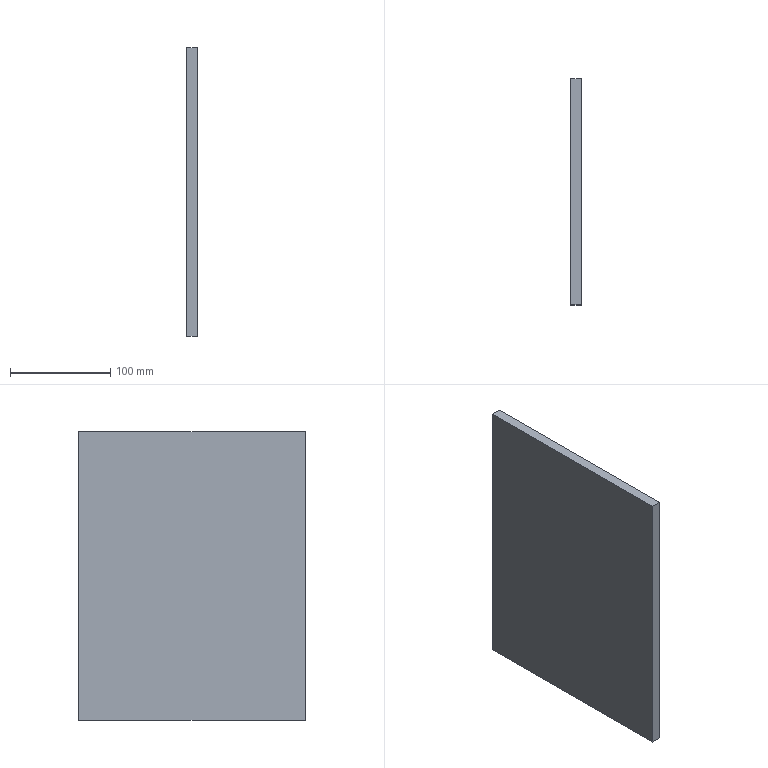Component | SolidWorks | Cover2-1 | 1 solid | 6 faces | box 10 x 226 x 288 mm | volume 650880 mm3 | plane 6 | material Plain Carbon Steel
STEP:
#1=COLOUR_RGB('',0.7922,0.8196,0.9333);
#2=FILL_AREA_STYLE_COLOUR('',#1);
#3=FILL_AREA_STYLE('',(#2));
#4=SURFACE_STYLE_FILL_AREA(#3);
#5=SURFACE_SIDE_STYLE('',(#4));
#6=SURFACE_STYLE_USAGE(.BOTH.,#5);
#7=PRESENTATION_STYLE_ASSIGNMENT((#6));
#8=CARTESIAN_POINT('',(88.212,53.911,76.893));
#9=VERTEX_POINT('',#8);
#10=CARTESIAN_POINT('',(88.212,53.911,65.555));
#11=VERTEX_POINT('',#10);
#12=CARTESIAN_POINT('',(88.212,53.911,65.555));
#13=DIRECTION('',(0.,-0.,-1.));
#14=VECTOR('',#13,39.37);
#15=LINE('',#12,#14);
#16=EDGE_CURVE('',#9,#11,#15,.T.);
#17=ORIENTED_EDGE('',*,*,#16,.F.);
#18=CARTESIAN_POINT('',(88.605,53.911,76.893));
#19=VERTEX_POINT('',#18);
#20=CARTESIAN_POINT('',(88.605,53.911,76.893));
#21=DIRECTION('',(-1.,-0.,0.));
#22=VECTOR('',#21,39.37);
#23=LINE('',#20,#22);
#24=EDGE_CURVE('',#19,#9,#23,.T.);
#25=ORIENTED_EDGE('',*,*,#24,.F.);
#26=CARTESIAN_POINT('',(88.605,53.911,65.555));
#27=VERTEX_POINT('',#26);
#28=CARTESIAN_POINT('',(88.605,53.911,65.555));
#29=DIRECTION('',(0.,-0.,-1.));
#30=VECTOR('',#29,39.37);
#31=LINE('',#28,#30);
#32=EDGE_CURVE('',#19,#27,#31,.T.);
#33=ORIENTED_EDGE('',*,*,#32,.T.);
#34=CARTESIAN_POINT('',(88.605,53.911,65.555));
#35=DIRECTION('',(-1.,-0.,0.));
#36=VECTOR('',#35,39.37);
#37=LINE('',#34,#36);
#38=EDGE_CURVE('',#27,#11,#37,.T.);
#39=ORIENTED_EDGE('',*,*,#38,.T.);
#40=EDGE_LOOP('',(#17,#25,#33,#39));
#41=FACE_OUTER_BOUND('',#40,.T.);
#42=CARTESIAN_POINT('',(88.605,53.911,65.555));
#43=DIRECTION('',(-0.,1.,-0.));
#44=DIRECTION('',(0.,-0.,-1.));
#45=AXIS2_PLACEMENT_3D('',#42,#43,#44);
#46=PLANE('',#45);
#47=ADVANCED_FACE('',(#41),#46,.T.);
#48=CARTESIAN_POINT('',(88.212,45.014,76.893));
#49=VERTEX_POINT('',#48);
#50=CARTESIAN_POINT('',(88.212,45.014,76.893));
#51=DIRECTION('',(-0.,1.,0.));
#52=VECTOR('',#51,39.37);
#53=LINE('',#50,#52);
#54=EDGE_CURVE('',#49,#9,#53,.T.);
#55=ORIENTED_EDGE('',*,*,#54,.F.);
#56=CARTESIAN_POINT('',(88.605,45.014,76.893));
#57=VERTEX_POINT('',#56);
#58=CARTESIAN_POINT('',(88.605,45.014,76.893));
#59=DIRECTION('',(-1.,-0.,0.));
#60=VECTOR('',#59,39.37);
#61=LINE('',#58,#60);
#62=EDGE_CURVE('',#57,#49,#61,.T.);
#63=ORIENTED_EDGE('',*,*,#62,.F.);
#64=CARTESIAN_POINT('',(88.605,45.014,76.893));
#65=DIRECTION('',(-0.,1.,0.));
#66=VECTOR('',#65,39.37);
#67=LINE('',#64,#66);
#68=EDGE_CURVE('',#57,#19,#67,.T.);
#69=ORIENTED_EDGE('',*,*,#68,.T.);
#70=ORIENTED_EDGE('',*,*,#24,.T.);
#71=EDGE_LOOP('',(#55,#63,#69,#70));
#72=FACE_OUTER_BOUND('',#71,.T.);
#73=CARTESIAN_POINT('',(88.605,45.014,76.893));
#74=DIRECTION('',(0.,0.,1.));
#75=DIRECTION('',(-0.,1.,0.));
#76=AXIS2_PLACEMENT_3D('',#73,#74,#75);
#77=PLANE('',#76);
#78=ADVANCED_FACE('',(#72),#77,.T.);
#79=CARTESIAN_POINT('',(88.212,45.014,65.555));
#80=VERTEX_POINT('',#79);
#81=CARTESIAN_POINT('',(88.212,45.014,65.555));
#82=DIRECTION('',(-0.,0.,1.));
#83=VECTOR('',#82,39.37);
#84=LINE('',#81,#83);
#85=EDGE_CURVE('',#80,#49,#84,.T.);
#86=ORIENTED_EDGE('',*,*,#85,.F.);
#87=CARTESIAN_POINT('',(88.605,45.014,65.555));
#88=VERTEX_POINT('',#87);
#89=CARTESIAN_POINT('',(88.605,45.014,65.555));
#90=DIRECTION('',(-1.,-0.,0.));
#91=VECTOR('',#90,39.37);
#92=LINE('',#89,#91);
#93=EDGE_CURVE('',#88,#80,#92,.T.);
#94=ORIENTED_EDGE('',*,*,#93,.F.);
#95=CARTESIAN_POINT('',(88.605,45.014,65.555));
#96=DIRECTION('',(-0.,0.,1.));
#97=VECTOR('',#96,39.37);
#98=LINE('',#95,#97);
#99=EDGE_CURVE('',#88,#57,#98,.T.);
#100=ORIENTED_EDGE('',*,*,#99,.T.);
#101=ORIENTED_EDGE('',*,*,#62,.T.);
#102=EDGE_LOOP('',(#86,#94,#100,#101));
#103=FACE_OUTER_BOUND('',#102,.T.);
#104=CARTESIAN_POINT('',(88.605,45.014,65.555));
#105=DIRECTION('',(0.,-1.,0.));
#106=DIRECTION('',(-0.,0.,1.));
#107=AXIS2_PLACEMENT_3D('',#104,#105,#106);
#108=PLANE('',#107);
#109=ADVANCED_FACE('',(#103),#108,.T.);
#110=CARTESIAN_POINT('',(88.212,45.014,65.555));
#111=DIRECTION('',(0.,-1.,0.));
#112=VECTOR('',#111,39.37);
#113=LINE('',#110,#112);
#114=EDGE_CURVE('',#11,#80,#113,.T.);
#115=ORIENTED_EDGE('',*,*,#114,.F.);
#116=ORIENTED_EDGE('',*,*,#38,.F.);
#117=CARTESIAN_POINT('',(88.605,45.014,65.555));
#118=DIRECTION('',(0.,-1.,0.));
#119=VECTOR('',#118,39.37);
#120=LINE('',#117,#119);
#121=EDGE_CURVE('',#27,#88,#120,.T.);
#122=ORIENTED_EDGE('',*,*,#121,.T.);
#123=ORIENTED_EDGE('',*,*,#93,.T.);
#124=EDGE_LOOP('',(#115,#116,#122,#123));
#125=FACE_OUTER_BOUND('',#124,.T.);
#126=CARTESIAN_POINT('',(88.605,45.014,65.555));
#127=DIRECTION('',(0.,0.,-1.));
#128=DIRECTION('',(0.,-1.,0.));
#129=AXIS2_PLACEMENT_3D('',#126,#127,#128);
#130=PLANE('',#129);
#131=ADVANCED_FACE('',(#125),#130,.T.);
#132=ORIENTED_EDGE('',*,*,#32,.F.);
#133=ORIENTED_EDGE('',*,*,#68,.F.);
#134=ORIENTED_EDGE('',*,*,#99,.F.);
#135=ORIENTED_EDGE('',*,*,#121,.F.);
#136=EDGE_LOOP('',(#132,#133,#134,#135));
#137=FACE_OUTER_BOUND('',#136,.T.);
#138=CARTESIAN_POINT('',(88.605,49.463,71.224));
#139=DIRECTION('',(-1.,-0.,0.));
#140=DIRECTION('',(0.,0.,1.));
#141=AXIS2_PLACEMENT_3D('',#138,#139,#140);
#142=PLANE('',#141);
#143=ADVANCED_FACE('',(#137),#142,.F.);
#144=ORIENTED_EDGE('',*,*,#16,.T.);
#145=ORIENTED_EDGE('',*,*,#114,.T.);
#146=ORIENTED_EDGE('',*,*,#85,.T.);
#147=ORIENTED_EDGE('',*,*,#54,.T.);
#148=EDGE_LOOP('',(#144,#145,#146,#147));
#149=FACE_OUTER_BOUND('',#148,.T.);
#150=CARTESIAN_POINT('',(88.212,49.463,71.224));
#151=DIRECTION('',(-1.,-0.,0.));
#152=DIRECTION('',(0.,0.,1.));
#153=AXIS2_PLACEMENT_3D('',#150,#151,#152);
#154=PLANE('',#153);
#155=ADVANCED_FACE('',(#149),#154,.T.);
#156=CLOSED_SHELL('',(#47,#78,#109,#131,#143,#155));
#157=MANIFOLD_SOLID_BREP('',#156);
#158=STYLED_ITEM('',(#7),#157);
#159=PRESENTATION_LAYER_ASSIGNMENT('','',(#158));
#160=(LENGTH_UNIT()NAMED_UNIT(*)SI_UNIT($,.METRE.));
#161=LENGTH_MEASURE_WITH_UNIT(LENGTH_MEASURE(0.0254),#160);
#162=DIMENSIONAL_EXPONENTS(1.,0.,0.,0.,0.,0.,0.);
#163=(CONVERSION_BASED_UNIT('',#161)LENGTH_UNIT()NAMED_UNIT(#162));
#164=UNCERTAINTY_MEASURE_WITH_UNIT(LENGTH_MEASURE(0.00001),#163,'','');
#165=(NAMED_UNIT(*)PLANE_ANGLE_UNIT()SI_UNIT($,.RADIAN.));
#166=(NAMED_UNIT(*)SI_UNIT($,.STERADIAN.)SOLID_ANGLE_UNIT());
#167=(GEOMETRIC_REPRESENTATION_CONTEXT(3)GLOBAL_UNCERTAINTY_ASSIGNED_CONTEXT((#164))GLOBAL_UNIT_ASSIGNED_CONTEXT((#163,#165,#166))REPRESENTATION_CONTEXT('',''));
#168=MECHANICAL_DESIGN_GEOMETRIC_PRESENTATION_REPRESENTATION('',(#158),#167);
#169=CARTESIAN_POINT('',(0.,0.,0.));
#170=DIRECTION('',(0.,0.,1.));
#171=DIRECTION('',(1.,0.,0.));
#172=AXIS2_PLACEMENT_3D('',#169,#170,#171);
#173=(LENGTH_UNIT()NAMED_UNIT(*)SI_UNIT($,.METRE.));
#174=LENGTH_MEASURE_WITH_UNIT(LENGTH_MEASURE(0.0254),#173);
#175=DIMENSIONAL_EXPONENTS(1.,0.,0.,0.,0.,0.,0.);
#176=(CONVERSION_BASED_UNIT('',#174)LENGTH_UNIT()NAMED_UNIT(#175));
#177=UNCERTAINTY_MEASURE_WITH_UNIT(LENGTH_MEASURE(0.00001),#176,'','');
#178=(NAMED_UNIT(*)PLANE_ANGLE_UNIT()SI_UNIT($,.RADIAN.));
#179=(NAMED_UNIT(*)SI_UNIT($,.STERADIAN.)SOLID_ANGLE_UNIT());
#180=(GEOMETRIC_REPRESENTATION_CONTEXT(3)GLOBAL_UNCERTAINTY_ASSIGNED_CONTEXT((#177))GLOBAL_UNIT_ASSIGNED_CONTEXT((#176,#178,#179))REPRESENTATION_CONTEXT('',''));
#181=ADVANCED_BREP_SHAPE_REPRESENTATION('',(#157,#172),#180);